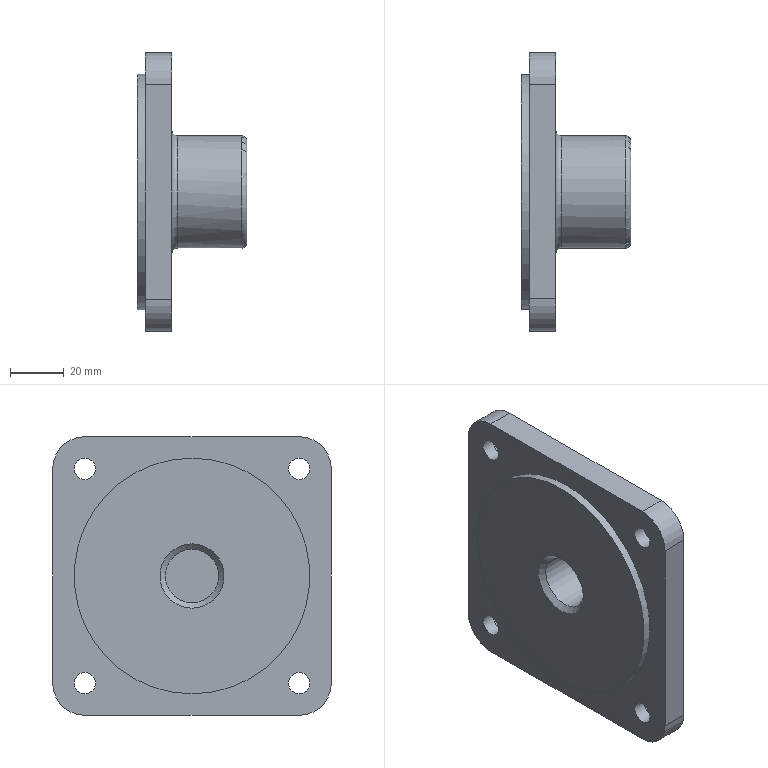Component | NX | PUMP_COVER | 1 solid | 33 faces | volume 150588 mm3 | cylinder 16 | plane 14 | torus 2 | cone 1 | commonest cylinder face diameters 24 x5 8 x4 12 x4 88 x1 42 x1 20 x1